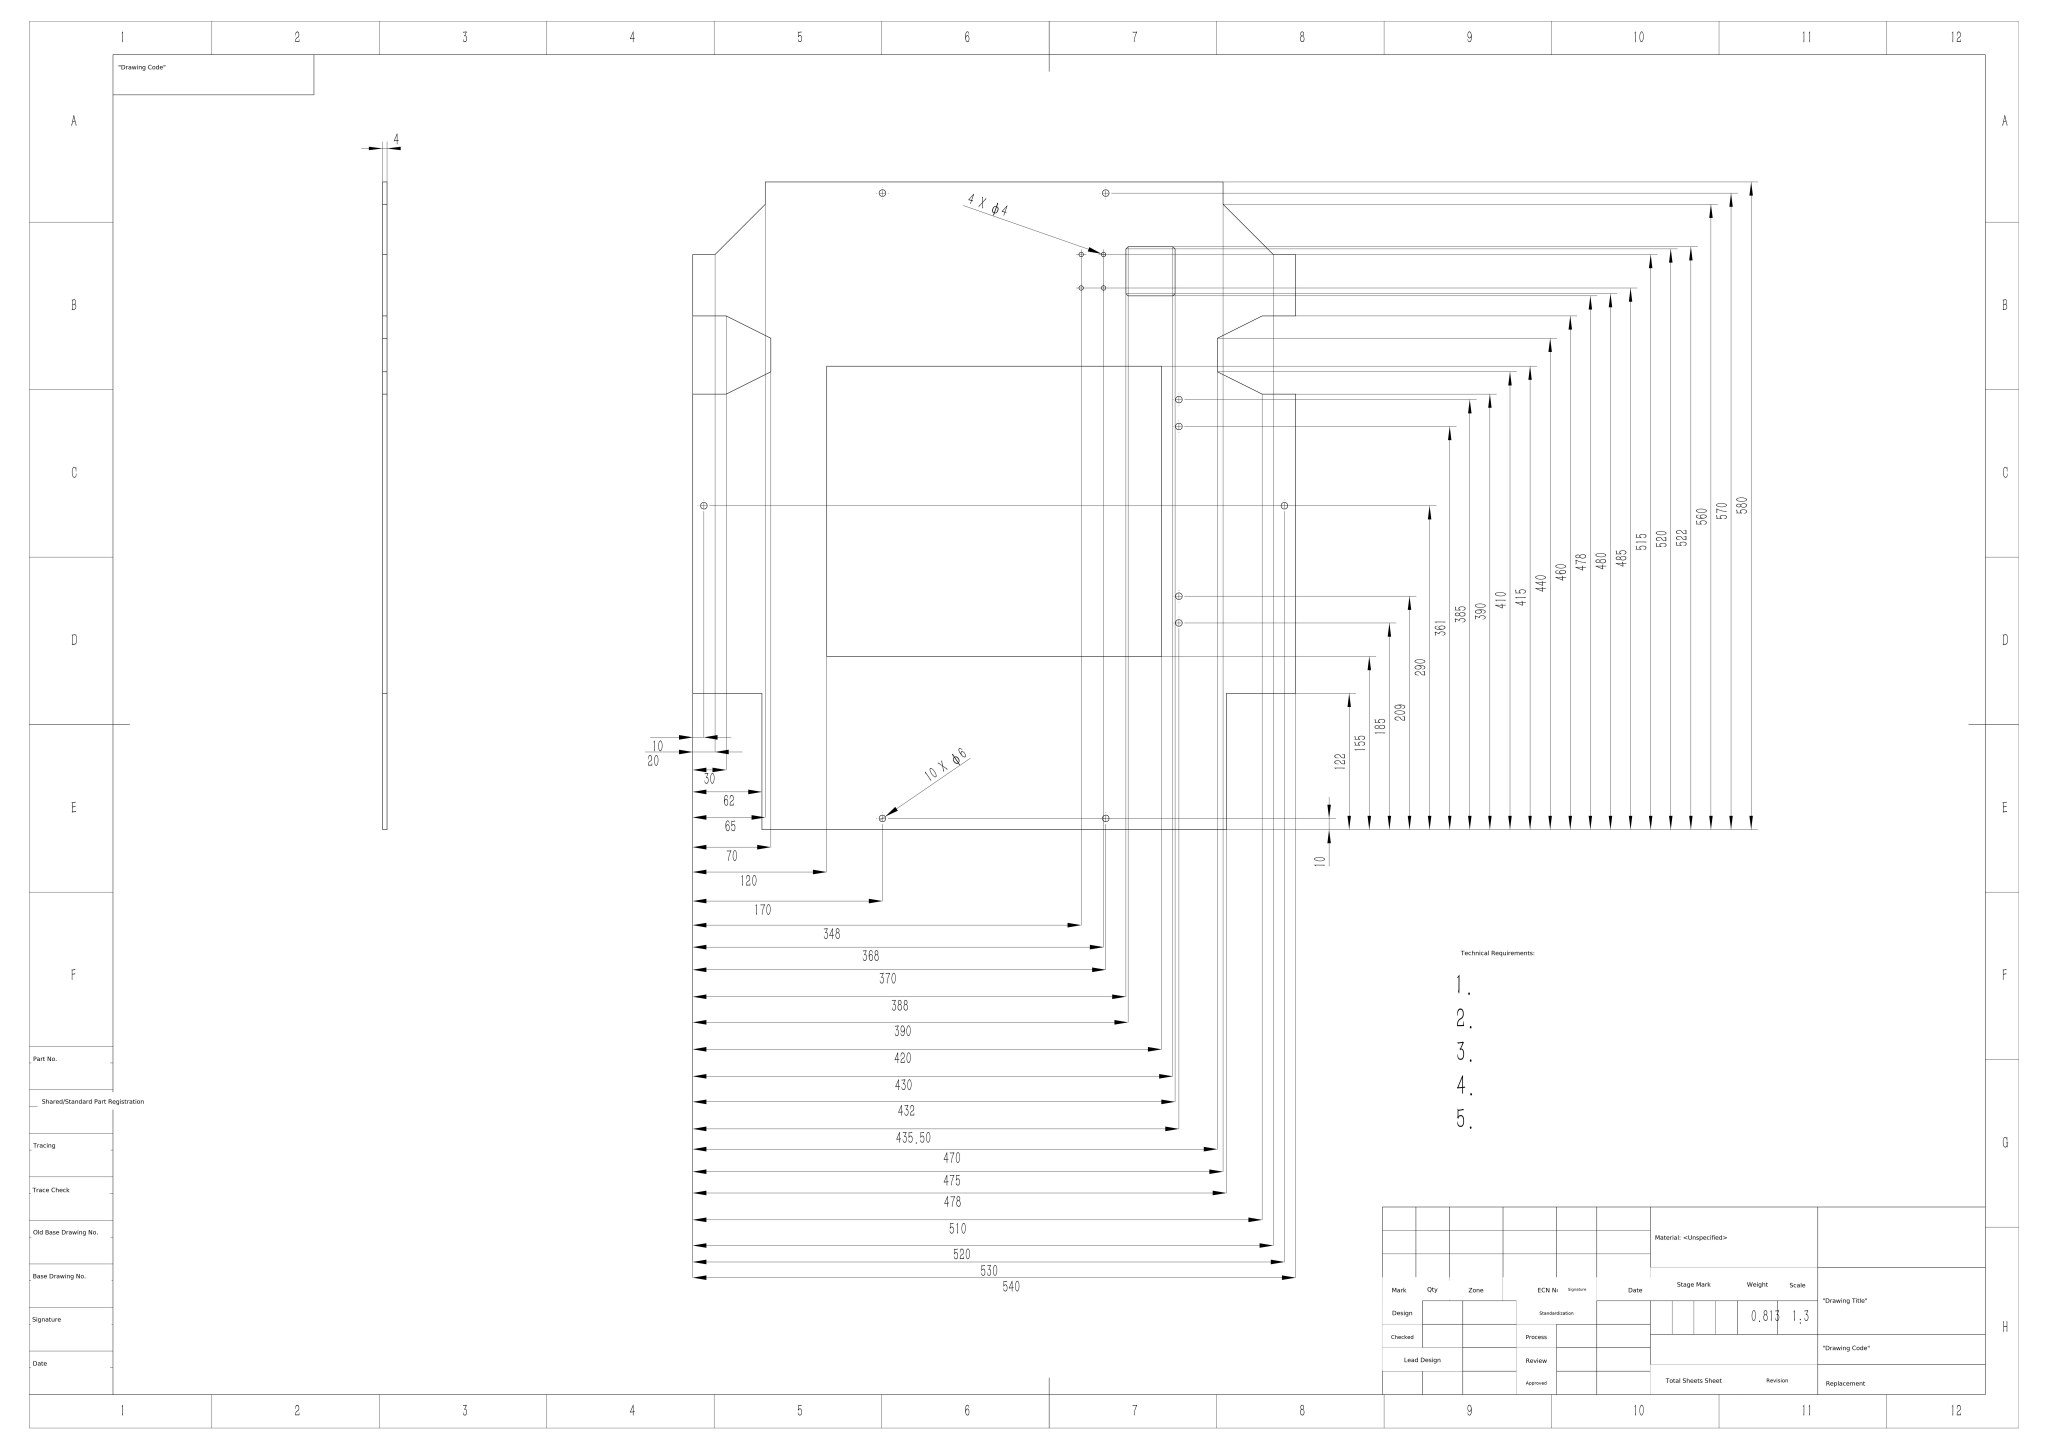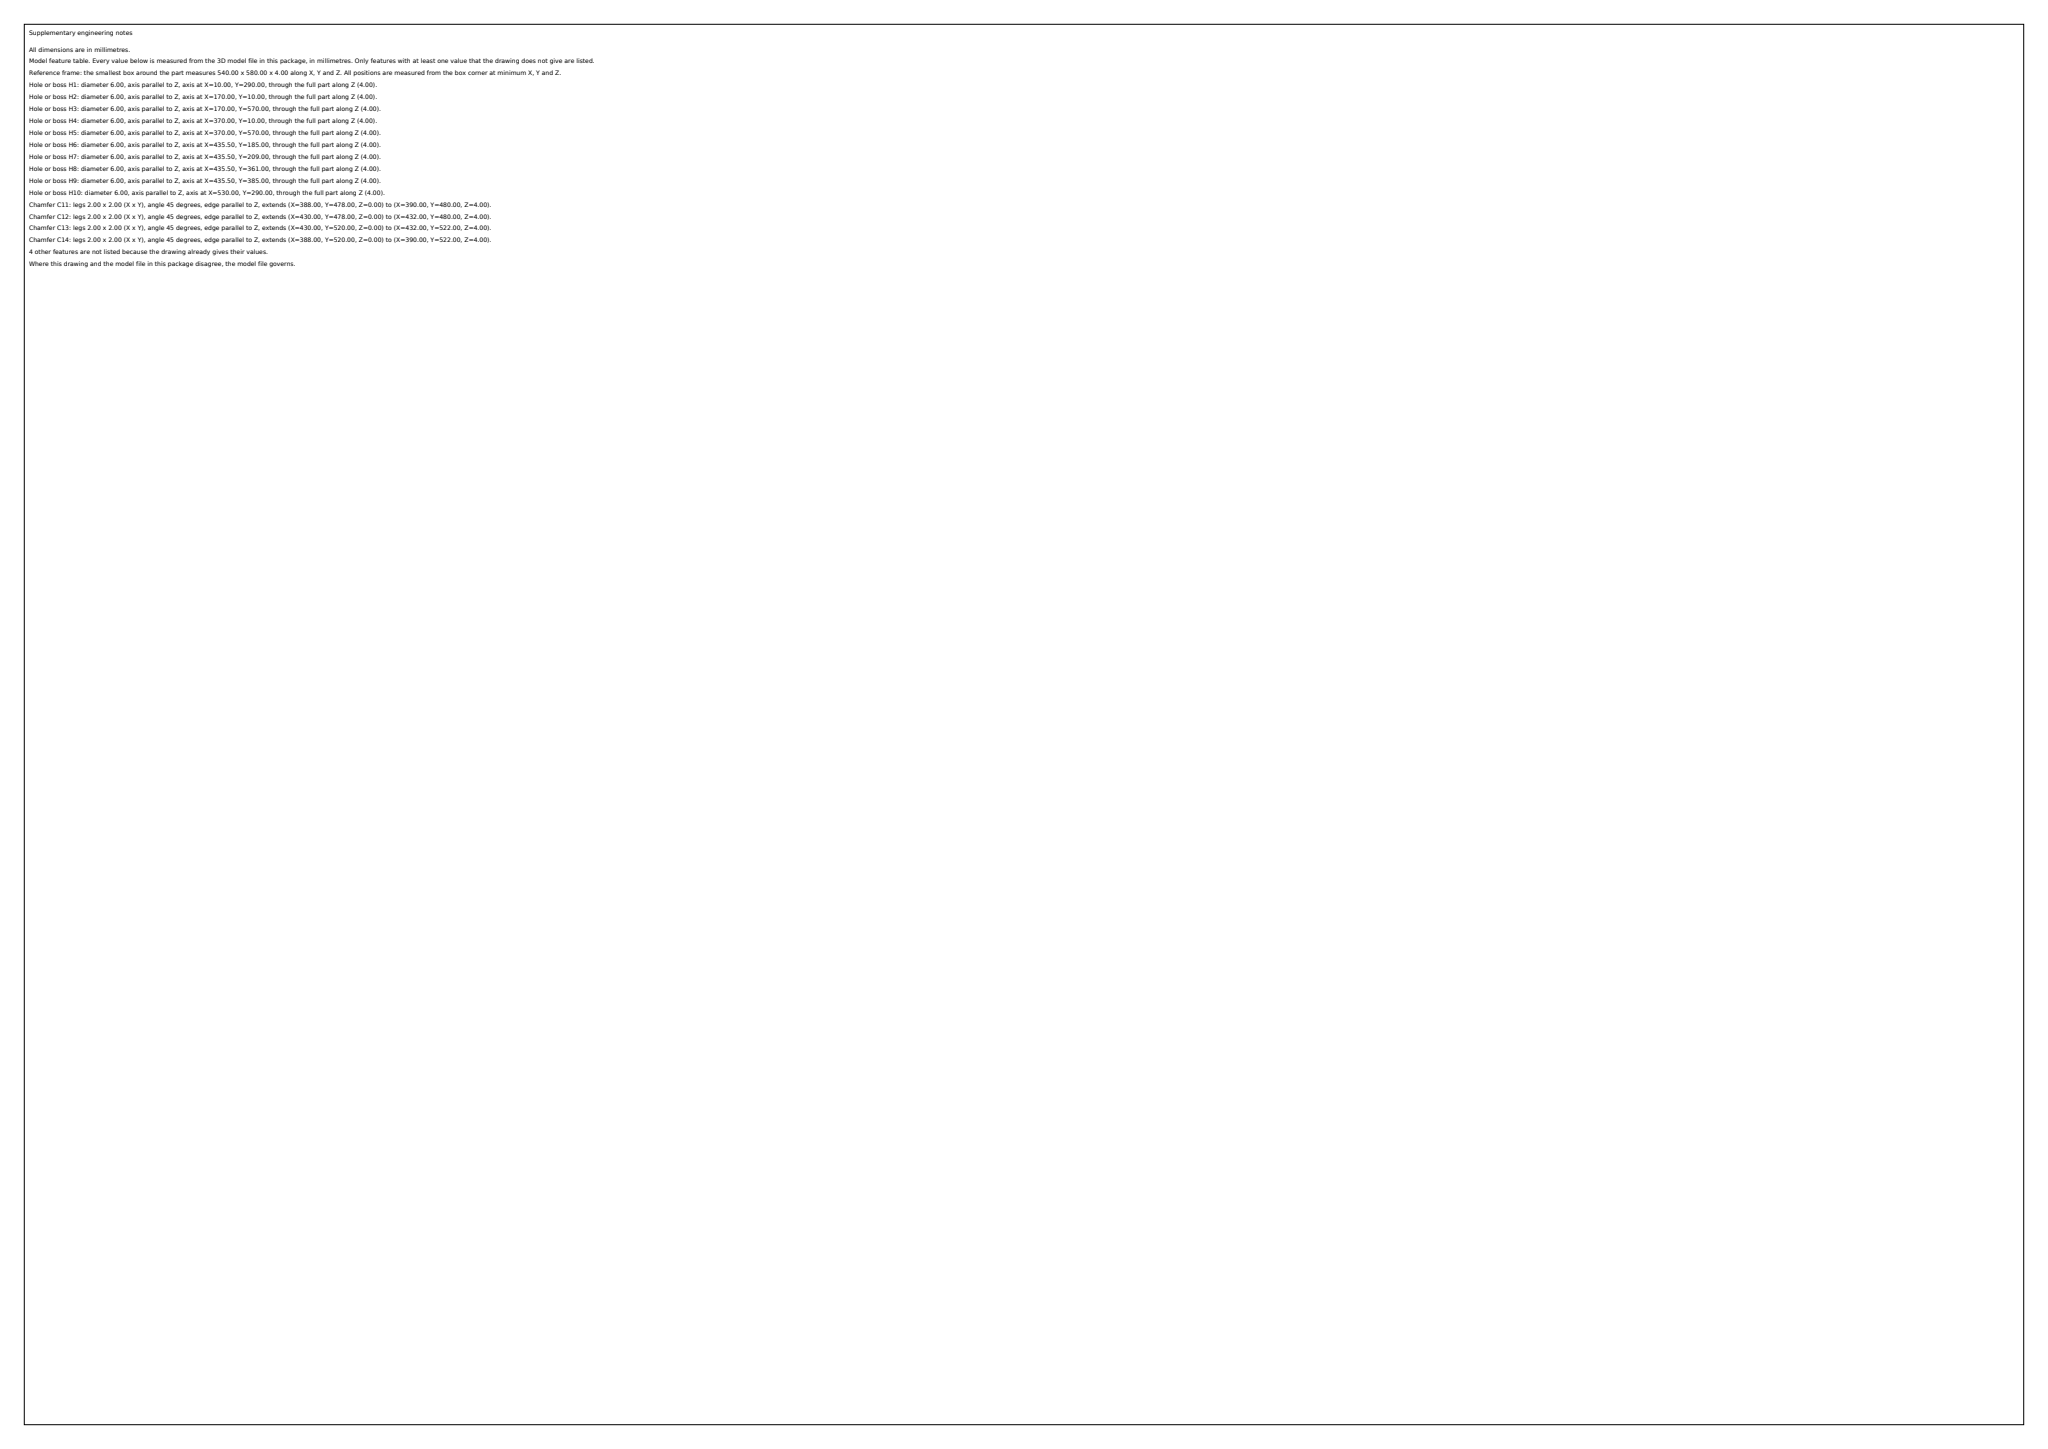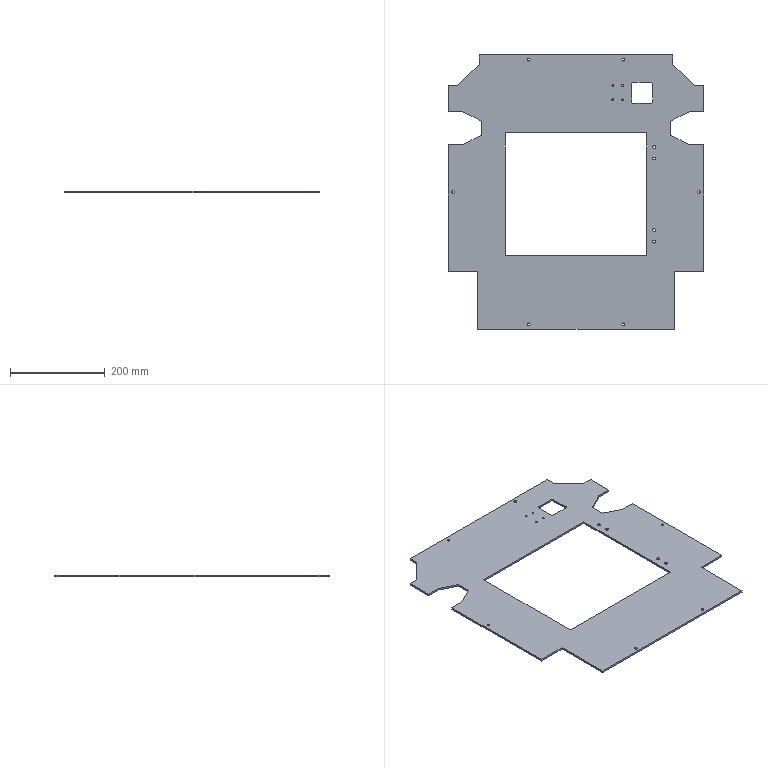Part | SolidWorks | mm | material <Unspecified> | 1 solid | 68 faces | box 540 x 580 x 4 mm | volume 812744 mm3 | plane 40 | cylinder 28 | commonest cylinder face diameters 6 x20 4 x8